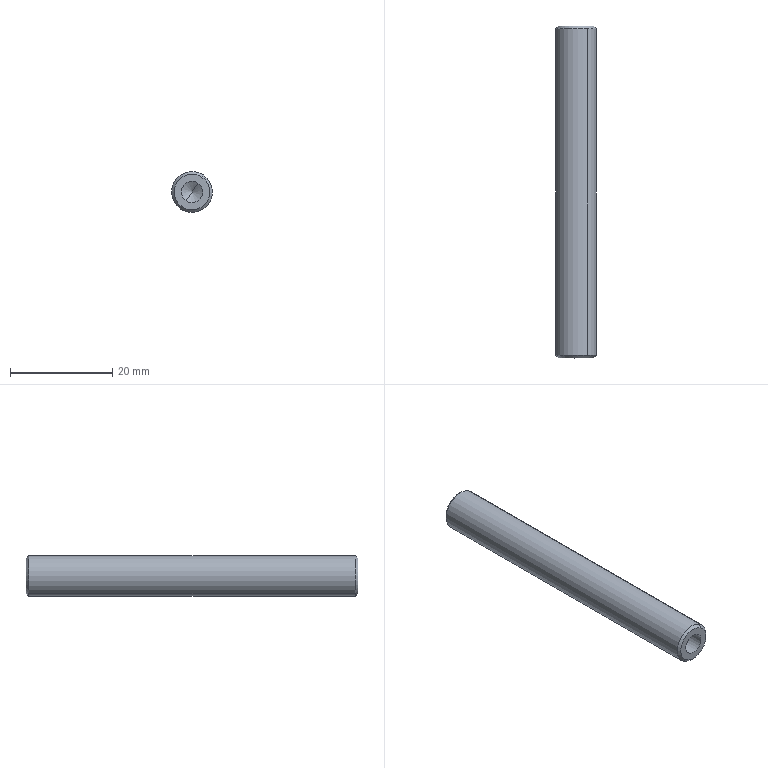Component | SolidWorks | WirePressingUnitGuidePost-1 | 1 solid | 12 faces | box 8 x 65 x 8 mm | volume 3084 mm3 | cone 6 | cylinder 4 | plane 2 | commonest cylinder face diameters 4.2 x2 8 x2
build123d program:
from build123d import *

# Parameters (mm, degrees)
SKETCH1_R             = 4
BOSS_EXTRUDE1_DEPTH   = 32.5
CHAMFER1_SIZE         = 0.5
M5_TAPPED_HOLE1_D     = 4.2
M5_TAPPED_HOLE1_DEPTH = 12.4
M5_TAPPED_HOLE1_TIP   = 1.262


with BuildPart() as part:
    # Sketch1 → Boss-Extrude1 (new, symmetric)
    with BuildSketch(Plane.XY):
        Circle(SKETCH1_R)
    extrude(amount=BOSS_EXTRUDE1_DEPTH, both=True)

    # Chamfer1
    chamfer1_edges = [part.edges().sort_by_distance(p)[0] for p in [
        (-4, 0, -32.5),
        (-4, 0, 32.5),
    ]]
    chamfer(chamfer1_edges, length=CHAMFER1_SIZE)

    # M5 Tapped Hole1
    with Locations(Plane.XY.offset(32.5)):
        with Locations((0, 0)):
            Hole(M5_TAPPED_HOLE1_D / 2, depth=M5_TAPPED_HOLE1_DEPTH)
            with Locations((0, 0, -(M5_TAPPED_HOLE1_DEPTH + M5_TAPPED_HOLE1_TIP / 2))):  # 118° drill point
                Cone(0, M5_TAPPED_HOLE1_D / 2, M5_TAPPED_HOLE1_TIP, mode=Mode.SUBTRACT)


solid = part.part

# Placed as in the assembly
solid = solid.moved(Location((-4.335, 71.668, -127.015), (90, 0, 0)))
STEP:
#1=COLOUR_RGB('',0.7922,0.8196,0.9333);
#2=FILL_AREA_STYLE_COLOUR('',#1);
#3=FILL_AREA_STYLE('',(#2));
#4=SURFACE_STYLE_FILL_AREA(#3);
#5=SURFACE_SIDE_STYLE('',(#4));
#6=SURFACE_STYLE_USAGE(.BOTH.,#5);
#7=PRESENTATION_STYLE_ASSIGNMENT((#6));
#8=CARTESIAN_POINT('',(-0.1249,2.03,-4.932));
#9=VERTEX_POINT('',#8);
#10=CARTESIAN_POINT('',(-0.2164,2.03,-5.069));
#11=VERTEX_POINT('',#10);
#12=CARTESIAN_POINT('',(-0.1707,2.03,-5.001));
#13=DIRECTION('',(0.,-1.,0.));
#14=DIRECTION('',(-0.5534,0.,-0.8329));
#15=AXIS2_PLACEMENT_3D('',#12,#13,#14);
#16=CIRCLE('',#15,0.08268);
#17=EDGE_CURVE('',#9,#11,#16,.T.);
#18=ORIENTED_EDGE('',*,*,#17,.F.);
#19=CARTESIAN_POINT('',(-0.1249,1.542,-4.932));
#20=VERTEX_POINT('',#19);
#21=CARTESIAN_POINT('',(-0.1249,1.542,-4.932));
#22=DIRECTION('',(0.,-1.,0.));
#23=VECTOR('',#22,39.37);
#24=LINE('',#21,#23);
#25=EDGE_CURVE('',#9,#20,#24,.T.);
#26=ORIENTED_EDGE('',*,*,#25,.T.);
#27=CARTESIAN_POINT('',(-0.2164,1.542,-5.069));
#28=VERTEX_POINT('',#27);
#29=CARTESIAN_POINT('',(-0.1707,1.542,-5.001));
#30=DIRECTION('',(0.,-1.,0.));
#31=DIRECTION('',(-0.5534,0.,-0.8329));
#32=AXIS2_PLACEMENT_3D('',#29,#30,#31);
#33=CIRCLE('',#32,0.08268);
#34=EDGE_CURVE('',#20,#28,#33,.T.);
#35=ORIENTED_EDGE('',*,*,#34,.T.);
#36=CARTESIAN_POINT('',(-0.2164,1.542,-5.069));
#37=DIRECTION('',(0.,-1.,0.));
#38=VECTOR('',#37,39.37);
#39=LINE('',#36,#38);
#40=EDGE_CURVE('',#11,#28,#39,.T.);
#41=ORIENTED_EDGE('',*,*,#40,.F.);
#42=EDGE_LOOP('',(#18,#26,#35,#41));
#43=FACE_OUTER_BOUND('',#42,.T.);
#44=CARTESIAN_POINT('',(-0.1707,1.542,-5.001));
#45=DIRECTION('',(0.,-1.,0.));
#46=DIRECTION('',(-0.5534,0.,-0.8329));
#47=AXIS2_PLACEMENT_3D('',#44,#45,#46);
#48=CYLINDRICAL_SURFACE('',#47,0.08268);
#49=ADVANCED_FACE('',(#43),#48,.F.);
#50=CARTESIAN_POINT('',(-0.1707,2.08,-5.001));
#51=VERTEX_POINT('',#50);
#52=CARTESIAN_POINT('',(-0.2164,2.03,-5.069));
#53=DIRECTION('',(-0.4744,-0.515,-0.7139));
#54=VECTOR('',#53,39.37);
#55=LINE('',#52,#54);
#56=EDGE_CURVE('',#51,#11,#55,.T.);
#57=ORIENTED_EDGE('',*,*,#56,.F.);
#58=CARTESIAN_POINT('',(-0.1249,2.03,-4.932));
#59=DIRECTION('',(0.4744,-0.515,0.7139));
#60=VECTOR('',#59,39.37);
#61=LINE('',#58,#60);
#62=EDGE_CURVE('',#51,#9,#61,.T.);
#63=ORIENTED_EDGE('',*,*,#62,.T.);
#64=ORIENTED_EDGE('',*,*,#17,.T.);
#65=EDGE_LOOP('',(#57,#63,#64));
#66=FACE_OUTER_BOUND('',#65,.T.);
#67=CARTESIAN_POINT('',(-0.1707,2.03,-5.001));
#68=DIRECTION('',(0.,-1.,0.));
#69=DIRECTION('',(-0.5534,0.,-0.8329));
#70=AXIS2_PLACEMENT_3D('',#67,#68,#69);
#71=CONICAL_SURFACE('',#70,0.08268,1.03);
#72=ADVANCED_FACE('',(#66),#71,.F.);
#73=CARTESIAN_POINT('',(-0.2469,1.542,-5.115));
#74=VERTEX_POINT('',#73);
#75=CARTESIAN_POINT('',(-0.09442,1.542,-4.886));
#76=VERTEX_POINT('',#75);
#77=CARTESIAN_POINT('',(-0.1707,1.542,-5.001));
#78=DIRECTION('',(0.,-1.,0.));
#79=DIRECTION('',(-0.5534,0.,-0.8329));
#80=AXIS2_PLACEMENT_3D('',#77,#78,#79);
#81=CIRCLE('',#80,0.1378);
#82=EDGE_CURVE('',#74,#76,#81,.T.);
#83=ORIENTED_EDGE('',*,*,#82,.F.);
#84=CARTESIAN_POINT('',(-0.2578,1.562,-5.132));
#85=VERTEX_POINT('',#84);
#86=CARTESIAN_POINT('',(-0.2469,1.542,-5.115));
#87=DIRECTION('',(-0.3913,0.7071,-0.589));
#88=VECTOR('',#87,39.37);
#89=LINE('',#86,#88);
#90=EDGE_CURVE('',#74,#85,#89,.T.);
#91=ORIENTED_EDGE('',*,*,#90,.T.);
#92=CARTESIAN_POINT('',(-0.08353,1.562,-4.869));
#93=VERTEX_POINT('',#92);
#94=CARTESIAN_POINT('',(-0.1707,1.562,-5.001));
#95=DIRECTION('',(0.,1.,0.));
#96=DIRECTION('',(-0.5534,0.,-0.8329));
#97=AXIS2_PLACEMENT_3D('',#94,#95,#96);
#98=CIRCLE('',#97,0.1575);
#99=EDGE_CURVE('',#93,#85,#98,.T.);
#100=ORIENTED_EDGE('',*,*,#99,.F.);
#101=CARTESIAN_POINT('',(-0.09442,1.542,-4.886));
#102=DIRECTION('',(0.3913,0.7071,0.589));
#103=VECTOR('',#102,39.37);
#104=LINE('',#101,#103);
#105=EDGE_CURVE('',#76,#93,#104,.T.);
#106=ORIENTED_EDGE('',*,*,#105,.F.);
#107=EDGE_LOOP('',(#83,#91,#100,#106));
#108=FACE_OUTER_BOUND('',#107,.T.);
#109=CARTESIAN_POINT('',(-0.1707,1.542,-5.001));
#110=DIRECTION('',(0.,1.,0.));
#111=DIRECTION('',(0.5534,0.,0.8329));
#112=AXIS2_PLACEMENT_3D('',#109,#110,#111);
#113=CONICAL_SURFACE('',#112,0.1378,0.7854);
#114=ADVANCED_FACE('',(#108),#113,.T.);
#115=CARTESIAN_POINT('',(-0.09442,4.101,-4.886));
#116=VERTEX_POINT('',#115);
#117=CARTESIAN_POINT('',(-0.2469,4.101,-5.115));
#118=VERTEX_POINT('',#117);
#119=CARTESIAN_POINT('',(-0.1707,4.101,-5.001));
#120=DIRECTION('',(0.,1.,0.));
#121=DIRECTION('',(-0.5534,0.,-0.8329));
#122=AXIS2_PLACEMENT_3D('',#119,#120,#121);
#123=CIRCLE('',#122,0.1378);
#124=EDGE_CURVE('',#116,#118,#123,.T.);
#125=ORIENTED_EDGE('',*,*,#124,.F.);
#126=CARTESIAN_POINT('',(-0.08353,4.081,-4.869));
#127=VERTEX_POINT('',#126);
#128=CARTESIAN_POINT('',(-0.08353,4.081,-4.869));
#129=DIRECTION('',(0.3913,-0.7071,0.589));
#130=VECTOR('',#129,39.37);
#131=LINE('',#128,#130);
#132=EDGE_CURVE('',#116,#127,#131,.T.);
#133=ORIENTED_EDGE('',*,*,#132,.T.);
#134=CARTESIAN_POINT('',(-0.2578,4.081,-5.132));
#135=VERTEX_POINT('',#134);
#136=CARTESIAN_POINT('',(-0.1707,4.081,-5.001));
#137=DIRECTION('',(0.,-1.,0.));
#138=DIRECTION('',(-0.5534,0.,-0.8329));
#139=AXIS2_PLACEMENT_3D('',#136,#137,#138);
#140=CIRCLE('',#139,0.1575);
#141=EDGE_CURVE('',#135,#127,#140,.T.);
#142=ORIENTED_EDGE('',*,*,#141,.F.);
#143=CARTESIAN_POINT('',(-0.2578,4.081,-5.132));
#144=DIRECTION('',(-0.3913,-0.7071,-0.589));
#145=VECTOR('',#144,39.37);
#146=LINE('',#143,#145);
#147=EDGE_CURVE('',#118,#135,#146,.T.);
#148=ORIENTED_EDGE('',*,*,#147,.F.);
#149=EDGE_LOOP('',(#125,#133,#142,#148));
#150=FACE_OUTER_BOUND('',#149,.T.);
#151=CARTESIAN_POINT('',(-0.1707,4.081,-5.001));
#152=DIRECTION('',(0.,-1.,0.));
#153=DIRECTION('',(-0.5534,0.,-0.8329));
#154=AXIS2_PLACEMENT_3D('',#151,#152,#153);
#155=CONICAL_SURFACE('',#154,0.1575,0.7854);
#156=ADVANCED_FACE('',(#150),#155,.T.);
#157=ORIENTED_EDGE('',*,*,#99,.T.);
#158=CARTESIAN_POINT('',(-0.2578,1.542,-5.132));
#159=DIRECTION('',(0.,1.,0.));
#160=VECTOR('',#159,39.37);
#161=LINE('',#158,#160);
#162=EDGE_CURVE('',#85,#135,#161,.T.);
#163=ORIENTED_EDGE('',*,*,#162,.T.);
#164=ORIENTED_EDGE('',*,*,#141,.T.);
#165=CARTESIAN_POINT('',(-0.08353,1.542,-4.869));
#166=DIRECTION('',(0.,1.,0.));
#167=VECTOR('',#166,39.37);
#168=LINE('',#165,#167);
#169=EDGE_CURVE('',#93,#127,#168,.T.);
#170=ORIENTED_EDGE('',*,*,#169,.F.);
#171=EDGE_LOOP('',(#157,#163,#164,#170));
#172=FACE_OUTER_BOUND('',#171,.T.);
#173=CARTESIAN_POINT('',(-0.1707,1.542,-5.001));
#174=DIRECTION('',(0.,1.,0.));
#175=DIRECTION('',(0.5534,0.,0.8329));
#176=AXIS2_PLACEMENT_3D('',#173,#174,#175);
#177=CYLINDRICAL_SURFACE('',#176,0.1575);
#178=ADVANCED_FACE('',(#172),#177,.T.);
#179=ORIENTED_EDGE('',*,*,#162,.F.);
#180=CARTESIAN_POINT('',(-0.1707,1.562,-5.001));
#181=DIRECTION('',(0.,1.,0.));
#182=DIRECTION('',(-0.5534,0.,-0.8329));
#183=AXIS2_PLACEMENT_3D('',#180,#181,#182);
#184=CIRCLE('',#183,0.1575);
#185=EDGE_CURVE('',#85,#93,#184,.T.);
#186=ORIENTED_EDGE('',*,*,#185,.T.);
#187=ORIENTED_EDGE('',*,*,#169,.T.);
#188=CARTESIAN_POINT('',(-0.1707,4.081,-5.001));
#189=DIRECTION('',(0.,-1.,0.));
#190=DIRECTION('',(-0.5534,0.,-0.8329));
#191=AXIS2_PLACEMENT_3D('',#188,#189,#190);
#192=CIRCLE('',#191,0.1575);
#193=EDGE_CURVE('',#127,#135,#192,.T.);
#194=ORIENTED_EDGE('',*,*,#193,.T.);
#195=EDGE_LOOP('',(#179,#186,#187,#194));
#196=FACE_OUTER_BOUND('',#195,.T.);
#197=CARTESIAN_POINT('',(-0.1707,1.542,-5.001));
#198=DIRECTION('',(0.,1.,0.));
#199=DIRECTION('',(0.5534,0.,0.8329));
#200=AXIS2_PLACEMENT_3D('',#197,#198,#199);
#201=CYLINDRICAL_SURFACE('',#200,0.1575);
#202=ADVANCED_FACE('',(#196),#201,.T.);
#203=CARTESIAN_POINT('',(-0.1707,1.542,-5.001));
#204=DIRECTION('',(0.,-1.,0.));
#205=DIRECTION('',(-0.5534,0.,-0.8329));
#206=AXIS2_PLACEMENT_3D('',#203,#204,#205);
#207=CIRCLE('',#206,0.08268);
#208=EDGE_CURVE('',#28,#20,#207,.T.);
#209=ORIENTED_EDGE('',*,*,#208,.F.);
#210=ORIENTED_EDGE('',*,*,#34,.F.);
#211=EDGE_LOOP('',(#209,#210));
#212=FACE_BOUND('',#211,.T.);
#213=CARTESIAN_POINT('',(-0.1707,1.542,-5.001));
#214=DIRECTION('',(0.,-1.,0.));
#215=DIRECTION('',(-0.5534,0.,-0.8329));
#216=AXIS2_PLACEMENT_3D('',#213,#214,#215);
#217=CIRCLE('',#216,0.1378);
#218=EDGE_CURVE('',#76,#74,#217,.T.);
#219=ORIENTED_EDGE('',*,*,#218,.T.);
#220=ORIENTED_EDGE('',*,*,#82,.T.);
#221=EDGE_LOOP('',(#219,#220));
#222=FACE_OUTER_BOUND('',#221,.T.);
#223=CARTESIAN_POINT('',(-0.1707,1.542,-5.001));
#224=DIRECTION('',(0.,-1.,0.));
#225=DIRECTION('',(-0.5534,0.,-0.8329));
#226=AXIS2_PLACEMENT_3D('',#223,#224,#225);
#227=PLANE('',#226);
#228=ADVANCED_FACE('',(#212,#222),#227,.T.);
#229=CARTESIAN_POINT('',(-0.1707,4.101,-5.001));
#230=DIRECTION('',(0.,1.,0.));
#231=DIRECTION('',(-0.5534,0.,-0.8329));
#232=AXIS2_PLACEMENT_3D('',#229,#230,#231);
#233=CIRCLE('',#232,0.1378);
#234=EDGE_CURVE('',#118,#116,#233,.T.);
#235=ORIENTED_EDGE('',*,*,#234,.T.);
#236=ORIENTED_EDGE('',*,*,#124,.T.);
#237=EDGE_LOOP('',(#235,#236));
#238=FACE_OUTER_BOUND('',#237,.T.);
#239=CARTESIAN_POINT('',(-0.1707,4.101,-5.001));
#240=DIRECTION('',(0.,-1.,0.));
#241=DIRECTION('',(-0.5534,0.,-0.8329));
#242=AXIS2_PLACEMENT_3D('',#239,#240,#241);
#243=PLANE('',#242);
#244=ADVANCED_FACE('',(#238),#243,.F.);
#245=ORIENTED_EDGE('',*,*,#132,.F.);
#246=ORIENTED_EDGE('',*,*,#234,.F.);
#247=ORIENTED_EDGE('',*,*,#147,.T.);
#248=ORIENTED_EDGE('',*,*,#193,.F.);
#249=EDGE_LOOP('',(#245,#246,#247,#248));
#250=FACE_OUTER_BOUND('',#249,.T.);
#251=CARTESIAN_POINT('',(-0.1707,4.081,-5.001));
#252=DIRECTION('',(0.,-1.,0.));
#253=DIRECTION('',(-0.5534,0.,-0.8329));
#254=AXIS2_PLACEMENT_3D('',#251,#252,#253);
#255=CONICAL_SURFACE('',#254,0.1575,0.7854);
#256=ADVANCED_FACE('',(#250),#255,.T.);
#257=ORIENTED_EDGE('',*,*,#90,.F.);
#258=ORIENTED_EDGE('',*,*,#218,.F.);
#259=ORIENTED_EDGE('',*,*,#105,.T.);
#260=ORIENTED_EDGE('',*,*,#185,.F.);
#261=EDGE_LOOP('',(#257,#258,#259,#260));
#262=FACE_OUTER_BOUND('',#261,.T.);
#263=CARTESIAN_POINT('',(-0.1707,1.542,-5.001));
#264=DIRECTION('',(0.,1.,0.));
#265=DIRECTION('',(0.5534,0.,0.8329));
#266=AXIS2_PLACEMENT_3D('',#263,#264,#265);
#267=CONICAL_SURFACE('',#266,0.1378,0.7854);
#268=ADVANCED_FACE('',(#262),#267,.T.);
#269=ORIENTED_EDGE('',*,*,#62,.F.);
#270=ORIENTED_EDGE('',*,*,#56,.T.);
#271=CARTESIAN_POINT('',(-0.1707,2.03,-5.001));
#272=DIRECTION('',(0.,-1.,0.));
#273=DIRECTION('',(-0.5534,0.,-0.8329));
#274=AXIS2_PLACEMENT_3D('',#271,#272,#273);
#275=CIRCLE('',#274,0.08268);
#276=EDGE_CURVE('',#11,#9,#275,.T.);
#277=ORIENTED_EDGE('',*,*,#276,.T.);
#278=EDGE_LOOP('',(#269,#270,#277));
#279=FACE_OUTER_BOUND('',#278,.T.);
#280=CARTESIAN_POINT('',(-0.1707,2.03,-5.001));
#281=DIRECTION('',(0.,-1.,0.));
#282=DIRECTION('',(-0.5534,0.,-0.8329));
#283=AXIS2_PLACEMENT_3D('',#280,#281,#282);
#284=CONICAL_SURFACE('',#283,0.08268,1.03);
#285=ADVANCED_FACE('',(#279),#284,.F.);
#286=ORIENTED_EDGE('',*,*,#25,.F.);
#287=ORIENTED_EDGE('',*,*,#276,.F.);
#288=ORIENTED_EDGE('',*,*,#40,.T.);
#289=ORIENTED_EDGE('',*,*,#208,.T.);
#290=EDGE_LOOP('',(#286,#287,#288,#289));
#291=FACE_OUTER_BOUND('',#290,.T.);
#292=CARTESIAN_POINT('',(-0.1707,1.542,-5.001));
#293=DIRECTION('',(0.,-1.,0.));
#294=DIRECTION('',(-0.5534,0.,-0.8329));
#295=AXIS2_PLACEMENT_3D('',#292,#293,#294);
#296=CYLINDRICAL_SURFACE('',#295,0.08268);
#297=ADVANCED_FACE('',(#291),#296,.F.);
#298=CLOSED_SHELL('',(#49,#72,#114,#156,#178,#202,#228,#244,#256,#268,#285,#297));
#299=MANIFOLD_SOLID_BREP('',#298);
#300=STYLED_ITEM('',(#7),#299);
#301=(LENGTH_UNIT()NAMED_UNIT(*)SI_UNIT($,.METRE.));
#302=LENGTH_MEASURE_WITH_UNIT(LENGTH_MEASURE(0.0254),#301);
#303=DIMENSIONAL_EXPONENTS(1.,0.,0.,0.,0.,0.,0.);
#304=(CONVERSION_BASED_UNIT('',#302)LENGTH_UNIT()NAMED_UNIT(#303));
#305=UNCERTAINTY_MEASURE_WITH_UNIT(LENGTH_MEASURE(0.00001),#304,'','');
#306=(NAMED_UNIT(*)PLANE_ANGLE_UNIT()SI_UNIT($,.RADIAN.));
#307=(NAMED_UNIT(*)SI_UNIT($,.STERADIAN.)SOLID_ANGLE_UNIT());
#308=(GEOMETRIC_REPRESENTATION_CONTEXT(3)GLOBAL_UNCERTAINTY_ASSIGNED_CONTEXT((#305))GLOBAL_UNIT_ASSIGNED_CONTEXT((#304,#306,#307))REPRESENTATION_CONTEXT('',''));
#309=MECHANICAL_DESIGN_GEOMETRIC_PRESENTATION_REPRESENTATION('',(#300),#308);
#310=CARTESIAN_POINT('',(0.,0.,0.));
#311=DIRECTION('',(0.,0.,1.));
#312=DIRECTION('',(1.,0.,0.));
#313=AXIS2_PLACEMENT_3D('',#310,#311,#312);
#314=(LENGTH_UNIT()NAMED_UNIT(*)SI_UNIT($,.METRE.));
#315=LENGTH_MEASURE_WITH_UNIT(LENGTH_MEASURE(0.0254),#314);
#316=DIMENSIONAL_EXPONENTS(1.,0.,0.,0.,0.,0.,0.);
#317=(CONVERSION_BASED_UNIT('',#315)LENGTH_UNIT()NAMED_UNIT(#316));
#318=UNCERTAINTY_MEASURE_WITH_UNIT(LENGTH_MEASURE(0.00001),#317,'','');
#319=(NAMED_UNIT(*)PLANE_ANGLE_UNIT()SI_UNIT($,.RADIAN.));
#320=(NAMED_UNIT(*)SI_UNIT($,.STERADIAN.)SOLID_ANGLE_UNIT());
#321=(GEOMETRIC_REPRESENTATION_CONTEXT(3)GLOBAL_UNCERTAINTY_ASSIGNED_CONTEXT((#318))GLOBAL_UNIT_ASSIGNED_CONTEXT((#317,#319,#320))REPRESENTATION_CONTEXT('',''));
#322=ADVANCED_BREP_SHAPE_REPRESENTATION('',(#299,#313),#321);
#323=PRESENTATION_LAYER_ASSIGNMENT('','',(#300));